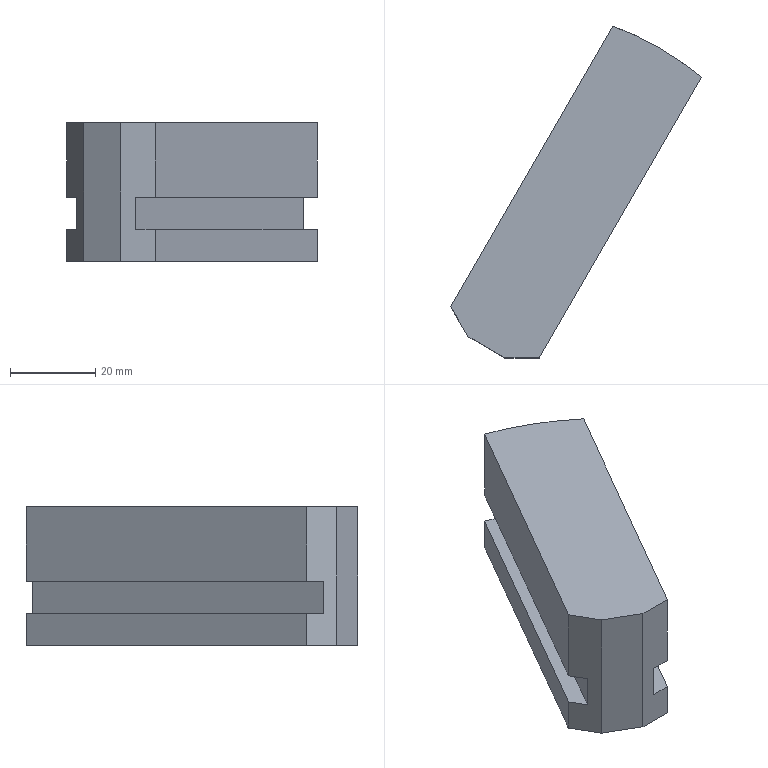Component | NX | JAW_2 | 1 solid | 16 faces | volume 57349 mm3 | plane 15 | cylinder 1 | commonest cylinder face diameters 140 x1